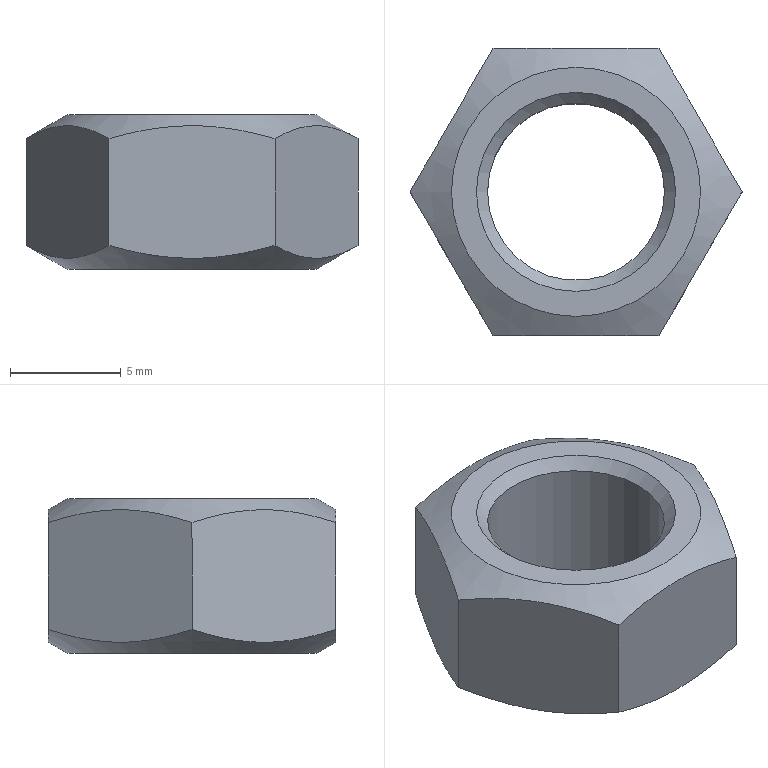Component | NX | NUT_M8 | 1 solid | 13 faces | volume 630 mm3 | plane 8 | cone 4 | cylinder 1 | commonest cylinder face diameters 8 x1